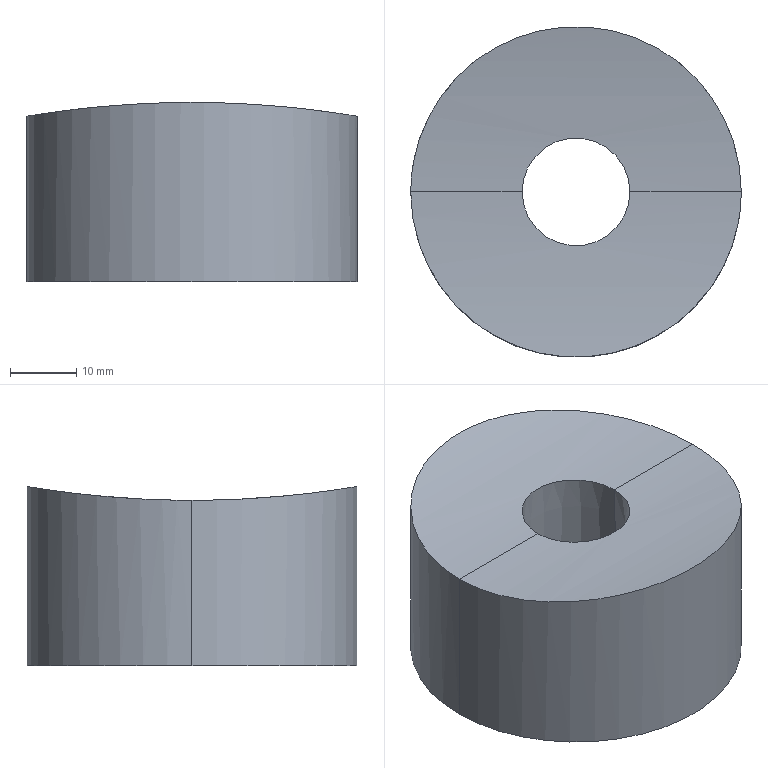Component | SolidWorks | JF21-80.1-1-3(_)-1-SOLID12-1 | 1 solid | 7 faces | box 50 x 50 x 27.1 mm | volume 44357 mm3 | cylinder 4 | cone 2 | plane 1 | commonest cylinder face diameters 300 x2 50 x2
STEP:
#1=CARTESIAN_POINT('',(8.34,-39.37,30.315));
#2=VERTEX_POINT('',#1);
#3=CARTESIAN_POINT('',(8.983,-39.37,30.315));
#4=VERTEX_POINT('',#3);
#5=CARTESIAN_POINT('',(8.34,-39.37,30.315));
#6=CARTESIAN_POINT('',(8.34,-39.391,30.315));
#7=CARTESIAN_POINT('',(8.342,-39.412,30.315));
#8=CARTESIAN_POINT('',(8.348,-39.443,30.315));
#9=CARTESIAN_POINT('',(8.351,-39.453,30.316));
#10=CARTESIAN_POINT('',(8.357,-39.473,30.316));
#11=CARTESIAN_POINT('',(8.361,-39.483,30.316));
#12=CARTESIAN_POINT('',(8.373,-39.512,30.317));
#13=CARTESIAN_POINT('',(8.383,-39.531,30.317));
#14=CARTESIAN_POINT('',(8.406,-39.566,30.318));
#15=CARTESIAN_POINT('',(8.42,-39.582,30.319));
#16=CARTESIAN_POINT('',(8.449,-39.612,30.32));
#17=CARTESIAN_POINT('',(8.465,-39.625,30.32));
#18=CARTESIAN_POINT('',(8.492,-39.643,30.321));
#19=CARTESIAN_POINT('',(8.501,-39.648,30.322));
#20=CARTESIAN_POINT('',(8.519,-39.658,30.322));
#21=CARTESIAN_POINT('',(8.538,-39.667,30.322));
#22=CARTESIAN_POINT('',(8.558,-39.674,30.323));
#23=CARTESIAN_POINT('',(8.578,-39.68,30.323));
#24=CARTESIAN_POINT('',(8.588,-39.683,30.323));
#25=CARTESIAN_POINT('',(8.619,-39.689,30.324));
#26=CARTESIAN_POINT('',(8.64,-39.691,30.324));
#27=CARTESIAN_POINT('',(8.682,-39.691,30.324));
#28=CARTESIAN_POINT('',(8.703,-39.689,30.324));
#29=CARTESIAN_POINT('',(8.745,-39.681,30.323));
#30=CARTESIAN_POINT('',(8.765,-39.675,30.323));
#31=CARTESIAN_POINT('',(8.794,-39.663,30.322));
#32=CARTESIAN_POINT('',(8.803,-39.658,30.322));
#33=CARTESIAN_POINT('',(8.822,-39.648,30.322));
#34=CARTESIAN_POINT('',(8.831,-39.643,30.321));
#35=CARTESIAN_POINT('',(8.857,-39.625,30.32));
#36=CARTESIAN_POINT('',(8.873,-39.612,30.32));
#37=CARTESIAN_POINT('',(8.903,-39.582,30.319));
#38=CARTESIAN_POINT('',(8.917,-39.566,30.318));
#39=CARTESIAN_POINT('',(8.934,-39.54,30.317));
#40=CARTESIAN_POINT('',(8.94,-39.531,30.317));
#41=CARTESIAN_POINT('',(8.95,-39.512,30.317));
#42=CARTESIAN_POINT('',(8.954,-39.503,30.316));
#43=CARTESIAN_POINT('',(8.966,-39.474,30.316));
#44=CARTESIAN_POINT('',(8.972,-39.454,30.316));
#45=CARTESIAN_POINT('',(8.981,-39.413,30.315));
#46=CARTESIAN_POINT('',(8.983,-39.391,30.315));
#47=CARTESIAN_POINT('',(8.983,-39.37,30.315));
#48=B_SPLINE_CURVE_WITH_KNOTS('',3,(#5,#6,#7,#8,#9,#10,#11,#12,#13,#14,#15,#16,#17,#18,#19,#20,#21,#22,#23,#24,#25,#26,#27,#28,#29,#30,#31,#32,#33,#34,#35,#36,#37,#38,#39,#40,#41,#42,#43,#44,#45,#46,#47),.UNSPECIFIED.,.F.,.F.,(4,2,2,2,2,2,2,2,1,2,2,2,2,2,2,2,2,2,2,2,2,4),(0.,0.001594,0.002391,0.003187,0.004781,0.006375,0.007968,0.008765,0.009562,0.01036,0.01116,0.01275,0.01434,0.01594,0.01673,0.01753,0.01912,0.02072,0.02151,0.02231,0.02391,0.0255),.UNSPECIFIED.);
#49=EDGE_CURVE('',#2,#4,#48,.T.);
#50=ORIENTED_EDGE('',*,*,#49,.T.);
#51=CARTESIAN_POINT('',(9.013,-39.37,29.331));
#52=VERTEX_POINT('',#51);
#53=CARTESIAN_POINT('',(9.013,-39.37,29.331));
#54=DIRECTION('',(-0.0312,-0.,0.9995));
#55=VECTOR('',#54,39.37);
#56=LINE('',#53,#55);
#57=EDGE_CURVE('',#52,#4,#56,.T.);
#58=ORIENTED_EDGE('',*,*,#57,.F.);
#59=CARTESIAN_POINT('',(8.309,-39.37,29.331));
#60=VERTEX_POINT('',#59);
#61=CARTESIAN_POINT('',(8.661,-39.37,29.331));
#62=DIRECTION('',(0.,0.,-1.));
#63=DIRECTION('',(-1.,0.,0.));
#64=AXIS2_PLACEMENT_3D('',#61,#62,#63);
#65=CIRCLE('',#64,0.352);
#66=EDGE_CURVE('',#52,#60,#65,.T.);
#67=ORIENTED_EDGE('',*,*,#66,.T.);
#68=CARTESIAN_POINT('',(8.309,-39.37,29.331));
#69=DIRECTION('',(0.0312,0.,0.9995));
#70=VECTOR('',#69,39.37);
#71=LINE('',#68,#70);
#72=EDGE_CURVE('',#60,#2,#71,.T.);
#73=ORIENTED_EDGE('',*,*,#72,.T.);
#74=EDGE_LOOP('',(#50,#58,#67,#73));
#75=FACE_OUTER_BOUND('',#74,.T.);
#76=CARTESIAN_POINT('',(8.661,-39.37,29.331));
#77=DIRECTION('',(0.,0.,-1.));
#78=DIRECTION('',(1.,0.,0.));
#79=AXIS2_PLACEMENT_3D('',#76,#77,#78);
#80=CONICAL_SURFACE('',#79,0.352,0.03121);
#81=ADVANCED_FACE('',(#75),#80,.F.);
#82=CARTESIAN_POINT('',(9.646,-39.37,30.315));
#83=VERTEX_POINT('',#82);
#84=CARTESIAN_POINT('',(7.677,-39.37,30.315));
#85=VERTEX_POINT('',#84);
#86=CARTESIAN_POINT('',(9.646,-39.37,30.315));
#87=CARTESIAN_POINT('',(9.646,-39.305,30.315));
#88=CARTESIAN_POINT('',(9.639,-39.241,30.316));
#89=CARTESIAN_POINT('',(9.62,-39.146,30.319));
#90=CARTESIAN_POINT('',(9.613,-39.115,30.32));
#91=CARTESIAN_POINT('',(9.594,-39.053,30.323));
#92=CARTESIAN_POINT('',(9.583,-39.023,30.325));
#93=CARTESIAN_POINT('',(9.546,-38.933,30.331));
#94=CARTESIAN_POINT('',(9.516,-38.877,30.335));
#95=CARTESIAN_POINT('',(9.471,-38.81,30.342));
#96=CARTESIAN_POINT('',(9.462,-38.797,30.343));
#97=CARTESIAN_POINT('',(9.442,-38.771,30.345));
#98=CARTESIAN_POINT('',(9.432,-38.758,30.347));
#99=CARTESIAN_POINT('',(9.402,-38.721,30.351));
#100=CARTESIAN_POINT('',(9.38,-38.697,30.353));
#101=CARTESIAN_POINT('',(9.312,-38.629,30.361));
#102=CARTESIAN_POINT('',(9.263,-38.588,30.367));
#103=CARTESIAN_POINT('',(9.195,-38.543,30.373));
#104=CARTESIAN_POINT('',(9.182,-38.534,30.374));
#105=CARTESIAN_POINT('',(9.154,-38.518,30.377));
#106=CARTESIAN_POINT('',(9.14,-38.51,30.378));
#107=CARTESIAN_POINT('',(9.097,-38.487,30.381));
#108=CARTESIAN_POINT('',(9.068,-38.473,30.383));
#109=CARTESIAN_POINT('',(9.009,-38.449,30.387));
#110=CARTESIAN_POINT('',(8.979,-38.438,30.389));
#111=CARTESIAN_POINT('',(8.933,-38.424,30.391));
#112=CARTESIAN_POINT('',(8.917,-38.42,30.392));
#113=CARTESIAN_POINT('',(8.886,-38.412,30.393));
#114=CARTESIAN_POINT('',(8.87,-38.408,30.394));
#115=CARTESIAN_POINT('',(8.79,-38.392,30.396));
#116=CARTESIAN_POINT('',(8.726,-38.386,30.398));
#117=CARTESIAN_POINT('',(8.63,-38.386,30.398));
#118=CARTESIAN_POINT('',(8.598,-38.387,30.397));
#119=CARTESIAN_POINT('',(8.549,-38.392,30.397));
#120=CARTESIAN_POINT('',(8.533,-38.394,30.396));
#121=CARTESIAN_POINT('',(8.501,-38.399,30.395));
#122=CARTESIAN_POINT('',(8.485,-38.402,30.395));
#123=CARTESIAN_POINT('',(8.406,-38.417,30.392));
#124=CARTESIAN_POINT('',(8.345,-38.436,30.389));
#125=CARTESIAN_POINT('',(8.255,-38.473,30.383));
#126=CARTESIAN_POINT('',(8.226,-38.487,30.381));
#127=CARTESIAN_POINT('',(8.169,-38.517,30.377));
#128=CARTESIAN_POINT('',(8.141,-38.534,30.374));
#129=CARTESIAN_POINT('',(8.088,-38.569,30.369));
#130=CARTESIAN_POINT('',(8.062,-38.588,30.367));
#131=CARTESIAN_POINT('',(8.013,-38.629,30.362));
#132=CARTESIAN_POINT('',(7.989,-38.651,30.359));
#133=CARTESIAN_POINT('',(7.92,-38.719,30.351));
#134=CARTESIAN_POINT('',(7.879,-38.769,30.345));
#135=CARTESIAN_POINT('',(7.826,-38.849,30.338));
#136=CARTESIAN_POINT('',(7.809,-38.876,30.336));
#137=CARTESIAN_POINT('',(7.786,-38.919,30.332));
#138=CARTESIAN_POINT('',(7.779,-38.934,30.331));
#139=CARTESIAN_POINT('',(7.765,-38.963,30.329));
#140=CARTESIAN_POINT('',(7.759,-38.978,30.328));
#141=CARTESIAN_POINT('',(7.728,-39.052,30.323));
#142=CARTESIAN_POINT('',(7.709,-39.113,30.32));
#143=CARTESIAN_POINT('',(7.69,-39.208,30.317));
#144=CARTESIAN_POINT('',(7.685,-39.24,30.316));
#145=CARTESIAN_POINT('',(7.679,-39.305,30.315));
#146=CARTESIAN_POINT('',(7.677,-39.338,30.315));
#147=CARTESIAN_POINT('',(7.677,-39.37,30.315));
#148=B_SPLINE_CURVE_WITH_KNOTS('',3,(#86,#87,#88,#89,#90,#91,#92,#93,#94,#95,#96,#97,#98,#99,#100,#101,#102,#103,#104,#105,#106,#107,#108,#109,#110,#111,#112,#113,#114,#115,#116,#117,#118,#119,#120,#121,#122,#123,#124,#125,#126,#127,#128,#129,#130,#131,#132,#133,#134,#135,#136,#137,#138,#139,#140,#141,#142,#143,#144,#145,#146,#147),.UNSPECIFIED.,.F.,.F.,(4,2,2,2,2,2,2,2,2,2,2,2,2,2,2,2,2,2,2,2,2,2,2,2,2,2,2,2,2,2,4),(0.,0.004892,0.007339,0.009785,0.01468,0.0159,0.01712,0.01957,0.02446,0.02569,0.02691,0.02935,0.0318,0.03302,0.03425,0.03914,0.04159,0.04281,0.04403,0.04892,0.05137,0.05382,0.05626,0.05871,0.0636,0.06605,0.06727,0.06849,0.07339,0.07583,0.07828),.UNSPECIFIED.);
#149=EDGE_CURVE('',#83,#85,#148,.T.);
#150=ORIENTED_EDGE('',*,*,#149,.T.);
#151=CARTESIAN_POINT('',(-15.748,-39.37,30.315));
#152=DIRECTION('',(1.,0.,0.));
#153=VECTOR('',#152,39.37);
#154=LINE('',#151,#153);
#155=EDGE_CURVE('',#85,#2,#154,.T.);
#156=ORIENTED_EDGE('',*,*,#155,.T.);
#157=CARTESIAN_POINT('',(8.983,-39.37,30.315));
#158=CARTESIAN_POINT('',(8.983,-39.349,30.315));
#159=CARTESIAN_POINT('',(8.981,-39.328,30.315));
#160=CARTESIAN_POINT('',(8.974,-39.297,30.315));
#161=CARTESIAN_POINT('',(8.972,-39.287,30.316));
#162=CARTESIAN_POINT('',(8.966,-39.267,30.316));
#163=CARTESIAN_POINT('',(8.962,-39.257,30.316));
#164=CARTESIAN_POINT('',(8.95,-39.228,30.317));
#165=CARTESIAN_POINT('',(8.94,-39.209,30.317));
#166=CARTESIAN_POINT('',(8.917,-39.174,30.318));
#167=CARTESIAN_POINT('',(8.903,-39.158,30.319));
#168=CARTESIAN_POINT('',(8.874,-39.128,30.32));
#169=CARTESIAN_POINT('',(8.858,-39.115,30.32));
#170=CARTESIAN_POINT('',(8.831,-39.097,30.321));
#171=CARTESIAN_POINT('',(8.822,-39.092,30.322));
#172=CARTESIAN_POINT('',(8.804,-39.082,30.322));
#173=CARTESIAN_POINT('',(8.785,-39.073,30.322));
#174=CARTESIAN_POINT('',(8.765,-39.066,30.323));
#175=CARTESIAN_POINT('',(8.745,-39.06,30.323));
#176=CARTESIAN_POINT('',(8.734,-39.057,30.323));
#177=CARTESIAN_POINT('',(8.703,-39.051,30.324));
#178=CARTESIAN_POINT('',(8.683,-39.049,30.324));
#179=CARTESIAN_POINT('',(8.641,-39.049,30.324));
#180=CARTESIAN_POINT('',(8.619,-39.051,30.324));
#181=CARTESIAN_POINT('',(8.578,-39.059,30.323));
#182=CARTESIAN_POINT('',(8.558,-39.065,30.323));
#183=CARTESIAN_POINT('',(8.529,-39.077,30.322));
#184=CARTESIAN_POINT('',(8.519,-39.082,30.322));
#185=CARTESIAN_POINT('',(8.501,-39.092,30.322));
#186=CARTESIAN_POINT('',(8.492,-39.097,30.321));
#187=CARTESIAN_POINT('',(8.466,-39.115,30.32));
#188=CARTESIAN_POINT('',(8.449,-39.128,30.32));
#189=CARTESIAN_POINT('',(8.419,-39.158,30.319));
#190=CARTESIAN_POINT('',(8.406,-39.174,30.318));
#191=CARTESIAN_POINT('',(8.389,-39.2,30.317));
#192=CARTESIAN_POINT('',(8.383,-39.209,30.317));
#193=CARTESIAN_POINT('',(8.373,-39.228,30.317));
#194=CARTESIAN_POINT('',(8.369,-39.237,30.316));
#195=CARTESIAN_POINT('',(8.357,-39.266,30.316));
#196=CARTESIAN_POINT('',(8.351,-39.286,30.316));
#197=CARTESIAN_POINT('',(8.342,-39.328,30.315));
#198=CARTESIAN_POINT('',(8.34,-39.349,30.315));
#199=CARTESIAN_POINT('',(8.34,-39.37,30.315));
#200=B_SPLINE_CURVE_WITH_KNOTS('',3,(#157,#158,#159,#160,#161,#162,#163,#164,#165,#166,#167,#168,#169,#170,#171,#172,#173,#174,#175,#176,#177,#178,#179,#180,#181,#182,#183,#184,#185,#186,#187,#188,#189,#190,#191,#192,#193,#194,#195,#196,#197,#198,#199),.UNSPECIFIED.,.F.,.F.,(4,2,2,2,2,2,2,2,1,2,2,2,2,2,2,2,2,2,2,2,2,4),(0.,0.001594,0.002391,0.003187,0.004781,0.006375,0.007968,0.008765,0.009562,0.01036,0.01116,0.01275,0.01434,0.01594,0.01673,0.01753,0.01912,0.02072,0.02151,0.02231,0.02391,0.0255),.UNSPECIFIED.);
#201=EDGE_CURVE('',#4,#2,#200,.T.);
#202=ORIENTED_EDGE('',*,*,#201,.F.);
#203=CARTESIAN_POINT('',(-15.748,-39.37,30.315));
#204=DIRECTION('',(1.,0.,0.));
#205=VECTOR('',#204,39.37);
#206=LINE('',#203,#205);
#207=EDGE_CURVE('',#4,#83,#206,.T.);
#208=ORIENTED_EDGE('',*,*,#207,.T.);
#209=EDGE_LOOP('',(#150,#156,#202,#208));
#210=FACE_OUTER_BOUND('',#209,.T.);
#211=CARTESIAN_POINT('',(-15.748,-39.37,36.22));
#212=DIRECTION('',(1.,0.,0.));
#213=DIRECTION('',(0.,0.,1.));
#214=AXIS2_PLACEMENT_3D('',#211,#212,#213);
#215=CYLINDRICAL_SURFACE('',#214,5.906);
#216=ADVANCED_FACE('',(#210),#215,.F.);
#217=ORIENTED_EDGE('',*,*,#149,.F.);
#218=CARTESIAN_POINT('',(9.646,-39.37,29.331));
#219=VERTEX_POINT('',#218);
#220=CARTESIAN_POINT('',(9.646,-39.37,30.709));
#221=DIRECTION('',(0.,0.,1.));
#222=VECTOR('',#221,39.37);
#223=LINE('',#220,#222);
#224=EDGE_CURVE('',#219,#83,#223,.T.);
#225=ORIENTED_EDGE('',*,*,#224,.F.);
#226=CARTESIAN_POINT('',(7.677,-39.37,29.331));
#227=VERTEX_POINT('',#226);
#228=CARTESIAN_POINT('',(8.661,-39.37,29.331));
#229=DIRECTION('',(0.,0.,1.));
#230=DIRECTION('',(1.,0.,0.));
#231=AXIS2_PLACEMENT_3D('',#228,#229,#230);
#232=CIRCLE('',#231,0.9843);
#233=EDGE_CURVE('',#219,#227,#232,.T.);
#234=ORIENTED_EDGE('',*,*,#233,.T.);
#235=CARTESIAN_POINT('',(7.677,-39.37,30.709));
#236=DIRECTION('',(0.,0.,1.));
#237=VECTOR('',#236,39.37);
#238=LINE('',#235,#237);
#239=EDGE_CURVE('',#227,#85,#238,.T.);
#240=ORIENTED_EDGE('',*,*,#239,.T.);
#241=EDGE_LOOP('',(#217,#225,#234,#240));
#242=FACE_OUTER_BOUND('',#241,.T.);
#243=CARTESIAN_POINT('',(8.661,-39.37,30.709));
#244=DIRECTION('',(0.,0.,-1.));
#245=DIRECTION('',(1.,0.,0.));
#246=AXIS2_PLACEMENT_3D('',#243,#244,#245);
#247=CYLINDRICAL_SURFACE('',#246,0.9843);
#248=ADVANCED_FACE('',(#242),#247,.T.);
#249=ORIENTED_EDGE('',*,*,#224,.T.);
#250=CARTESIAN_POINT('',(7.677,-39.37,30.315));
#251=CARTESIAN_POINT('',(7.677,-39.435,30.315));
#252=CARTESIAN_POINT('',(7.684,-39.499,30.316));
#253=CARTESIAN_POINT('',(7.702,-39.594,30.319));
#254=CARTESIAN_POINT('',(7.71,-39.625,30.32));
#255=CARTESIAN_POINT('',(7.729,-39.687,30.323));
#256=CARTESIAN_POINT('',(7.74,-39.718,30.325));
#257=CARTESIAN_POINT('',(7.777,-39.807,30.331));
#258=CARTESIAN_POINT('',(7.807,-39.863,30.335));
#259=CARTESIAN_POINT('',(7.852,-39.93,30.342));
#260=CARTESIAN_POINT('',(7.861,-39.943,30.343));
#261=CARTESIAN_POINT('',(7.88,-39.969,30.345));
#262=CARTESIAN_POINT('',(7.89,-39.982,30.347));
#263=CARTESIAN_POINT('',(7.921,-40.02,30.351));
#264=CARTESIAN_POINT('',(7.943,-40.043,30.353));
#265=CARTESIAN_POINT('',(8.011,-40.111,30.361));
#266=CARTESIAN_POINT('',(8.06,-40.152,30.367));
#267=CARTESIAN_POINT('',(8.127,-40.197,30.373));
#268=CARTESIAN_POINT('',(8.141,-40.206,30.374));
#269=CARTESIAN_POINT('',(8.169,-40.222,30.377));
#270=CARTESIAN_POINT('',(8.183,-40.23,30.378));
#271=CARTESIAN_POINT('',(8.225,-40.253,30.381));
#272=CARTESIAN_POINT('',(8.254,-40.267,30.383));
#273=CARTESIAN_POINT('',(8.314,-40.291,30.387));
#274=CARTESIAN_POINT('',(8.344,-40.302,30.389));
#275=CARTESIAN_POINT('',(8.39,-40.316,30.391));
#276=CARTESIAN_POINT('',(8.406,-40.321,30.392));
#277=CARTESIAN_POINT('',(8.437,-40.329,30.393));
#278=CARTESIAN_POINT('',(8.453,-40.332,30.394));
#279=CARTESIAN_POINT('',(8.532,-40.348,30.396));
#280=CARTESIAN_POINT('',(8.596,-40.354,30.398));
#281=CARTESIAN_POINT('',(8.693,-40.354,30.398));
#282=CARTESIAN_POINT('',(8.725,-40.353,30.397));
#283=CARTESIAN_POINT('',(8.774,-40.348,30.397));
#284=CARTESIAN_POINT('',(8.79,-40.346,30.396));
#285=CARTESIAN_POINT('',(8.822,-40.341,30.395));
#286=CARTESIAN_POINT('',(8.838,-40.339,30.395));
#287=CARTESIAN_POINT('',(8.917,-40.323,30.392));
#288=CARTESIAN_POINT('',(8.978,-40.304,30.389));
#289=CARTESIAN_POINT('',(9.067,-40.267,30.383));
#290=CARTESIAN_POINT('',(9.097,-40.253,30.381));
#291=CARTESIAN_POINT('',(9.154,-40.223,30.377));
#292=CARTESIAN_POINT('',(9.181,-40.206,30.374));
#293=CARTESIAN_POINT('',(9.235,-40.171,30.369));
#294=CARTESIAN_POINT('',(9.26,-40.152,30.367));
#295=CARTESIAN_POINT('',(9.31,-40.111,30.362));
#296=CARTESIAN_POINT('',(9.334,-40.089,30.359));
#297=CARTESIAN_POINT('',(9.403,-40.021,30.351));
#298=CARTESIAN_POINT('',(9.443,-39.971,30.345));
#299=CARTESIAN_POINT('',(9.497,-39.891,30.338));
#300=CARTESIAN_POINT('',(9.514,-39.864,30.336));
#301=CARTESIAN_POINT('',(9.536,-39.821,30.332));
#302=CARTESIAN_POINT('',(9.544,-39.807,30.331));
#303=CARTESIAN_POINT('',(9.558,-39.777,30.329));
#304=CARTESIAN_POINT('',(9.564,-39.762,30.328));
#305=CARTESIAN_POINT('',(9.595,-39.688,30.323));
#306=CARTESIAN_POINT('',(9.614,-39.627,30.32));
#307=CARTESIAN_POINT('',(9.633,-39.532,30.317));
#308=CARTESIAN_POINT('',(9.638,-39.5,30.316));
#309=CARTESIAN_POINT('',(9.644,-39.435,30.315));
#310=CARTESIAN_POINT('',(9.646,-39.403,30.315));
#311=CARTESIAN_POINT('',(9.646,-39.37,30.315));
#312=B_SPLINE_CURVE_WITH_KNOTS('',3,(#250,#251,#252,#253,#254,#255,#256,#257,#258,#259,#260,#261,#262,#263,#264,#265,#266,#267,#268,#269,#270,#271,#272,#273,#274,#275,#276,#277,#278,#279,#280,#281,#282,#283,#284,#285,#286,#287,#288,#289,#290,#291,#292,#293,#294,#295,#296,#297,#298,#299,#300,#301,#302,#303,#304,#305,#306,#307,#308,#309,#310,#311),.UNSPECIFIED.,.F.,.F.,(4,2,2,2,2,2,2,2,2,2,2,2,2,2,2,2,2,2,2,2,2,2,2,2,2,2,2,2,2,2,4),(0.,0.004892,0.007339,0.009785,0.01468,0.0159,0.01712,0.01957,0.02446,0.02569,0.02691,0.02935,0.0318,0.03302,0.03425,0.03914,0.04159,0.04281,0.04403,0.04892,0.05137,0.05382,0.05626,0.05871,0.0636,0.06605,0.06727,0.06849,0.07339,0.07583,0.07828),.UNSPECIFIED.);
#313=EDGE_CURVE('',#85,#83,#312,.T.);
#314=ORIENTED_EDGE('',*,*,#313,.F.);
#315=ORIENTED_EDGE('',*,*,#239,.F.);
#316=CARTESIAN_POINT('',(8.661,-39.37,29.331));
#317=DIRECTION('',(0.,0.,1.));
#318=DIRECTION('',(1.,0.,0.));
#319=AXIS2_PLACEMENT_3D('',#316,#317,#318);
#320=CIRCLE('',#319,0.9843);
#321=EDGE_CURVE('',#227,#219,#320,.T.);
#322=ORIENTED_EDGE('',*,*,#321,.T.);
#323=EDGE_LOOP('',(#249,#314,#315,#322));
#324=FACE_OUTER_BOUND('',#323,.T.);
#325=CARTESIAN_POINT('',(8.661,-39.37,30.709));
#326=DIRECTION('',(0.,0.,-1.));
#327=DIRECTION('',(1.,0.,0.));
#328=AXIS2_PLACEMENT_3D('',#325,#326,#327);
#329=CYLINDRICAL_SURFACE('',#328,0.9843);
#330=ADVANCED_FACE('',(#324),#329,.T.);
#331=CARTESIAN_POINT('',(8.661,-39.37,29.331));
#332=DIRECTION('',(0.,0.,-1.));
#333=DIRECTION('',(-1.,0.,0.));
#334=AXIS2_PLACEMENT_3D('',#331,#332,#333);
#335=CIRCLE('',#334,0.352);
#336=EDGE_CURVE('',#60,#52,#335,.T.);
#337=ORIENTED_EDGE('',*,*,#336,.F.);
#338=ORIENTED_EDGE('',*,*,#66,.F.);
#339=EDGE_LOOP('',(#337,#338));
#340=FACE_BOUND('',#339,.T.);
#341=ORIENTED_EDGE('',*,*,#321,.F.);
#342=ORIENTED_EDGE('',*,*,#233,.F.);
#343=EDGE_LOOP('',(#341,#342));
#344=FACE_OUTER_BOUND('',#343,.T.);
#345=CARTESIAN_POINT('',(8.661,-39.37,29.331));
#346=DIRECTION('',(0.,0.,1.));
#347=DIRECTION('',(-1.,0.,0.));
#348=AXIS2_PLACEMENT_3D('',#345,#346,#347);
#349=PLANE('',#348);
#350=ADVANCED_FACE('',(#340,#344),#349,.F.);
#351=ORIENTED_EDGE('',*,*,#155,.F.);
#352=ORIENTED_EDGE('',*,*,#313,.T.);
#353=ORIENTED_EDGE('',*,*,#207,.F.);
#354=ORIENTED_EDGE('',*,*,#49,.F.);
#355=EDGE_LOOP('',(#351,#352,#353,#354));
#356=FACE_OUTER_BOUND('',#355,.T.);
#357=CARTESIAN_POINT('',(-15.748,-39.37,36.22));
#358=DIRECTION('',(1.,0.,0.));
#359=DIRECTION('',(0.,0.,1.));
#360=AXIS2_PLACEMENT_3D('',#357,#358,#359);
#361=CYLINDRICAL_SURFACE('',#360,5.906);
#362=ADVANCED_FACE('',(#356),#361,.F.);
#363=ORIENTED_EDGE('',*,*,#57,.T.);
#364=ORIENTED_EDGE('',*,*,#201,.T.);
#365=ORIENTED_EDGE('',*,*,#72,.F.);
#366=ORIENTED_EDGE('',*,*,#336,.T.);
#367=EDGE_LOOP('',(#363,#364,#365,#366));
#368=FACE_OUTER_BOUND('',#367,.T.);
#369=CARTESIAN_POINT('',(8.661,-39.37,29.331));
#370=DIRECTION('',(0.,0.,-1.));
#371=DIRECTION('',(1.,0.,0.));
#372=AXIS2_PLACEMENT_3D('',#369,#370,#371);
#373=CONICAL_SURFACE('',#372,0.352,0.03121);
#374=ADVANCED_FACE('',(#368),#373,.F.);
#375=CLOSED_SHELL('',(#81,#216,#248,#330,#350,#362,#374));
#376=MANIFOLD_SOLID_BREP('',#375);
#377=CARTESIAN_POINT('',(0.,0.,0.));
#378=DIRECTION('',(0.,0.,1.));
#379=DIRECTION('',(1.,0.,0.));
#380=AXIS2_PLACEMENT_3D('',#377,#378,#379);
#381=(LENGTH_UNIT()NAMED_UNIT(*)SI_UNIT($,.METRE.));
#382=LENGTH_MEASURE_WITH_UNIT(LENGTH_MEASURE(0.0254),#381);
#383=DIMENSIONAL_EXPONENTS(1.,0.,0.,0.,0.,0.,0.);
#384=(CONVERSION_BASED_UNIT('',#382)LENGTH_UNIT()NAMED_UNIT(#383));
#385=UNCERTAINTY_MEASURE_WITH_UNIT(LENGTH_MEASURE(0.00001),#384,'','');
#386=(NAMED_UNIT(*)PLANE_ANGLE_UNIT()SI_UNIT($,.RADIAN.));
#387=(NAMED_UNIT(*)SI_UNIT($,.STERADIAN.)SOLID_ANGLE_UNIT());
#388=(GEOMETRIC_REPRESENTATION_CONTEXT(3)GLOBAL_UNCERTAINTY_ASSIGNED_CONTEXT((#385))GLOBAL_UNIT_ASSIGNED_CONTEXT((#384,#386,#387))REPRESENTATION_CONTEXT('',''));
#389=ADVANCED_BREP_SHAPE_REPRESENTATION('',(#376,#380),#388);
#390=COLOUR_RGB('',0.7922,0.8196,0.9333);
#391=FILL_AREA_STYLE_COLOUR('',#390);
#392=FILL_AREA_STYLE('',(#391));
#393=SURFACE_STYLE_FILL_AREA(#392);
#394=SURFACE_SIDE_STYLE('',(#393));
#395=SURFACE_STYLE_USAGE(.BOTH.,#394);
#396=PRESENTATION_STYLE_ASSIGNMENT((#395));
#397=STYLED_ITEM('',(#396),#376);
#398=PRESENTATION_LAYER_ASSIGNMENT('','',(#397));
#399=(LENGTH_UNIT()NAMED_UNIT(*)SI_UNIT($,.METRE.));
#400=LENGTH_MEASURE_WITH_UNIT(LENGTH_MEASURE(0.0254),#399);
#401=DIMENSIONAL_EXPONENTS(1.,0.,0.,0.,0.,0.,0.);
#402=(CONVERSION_BASED_UNIT('',#400)LENGTH_UNIT()NAMED_UNIT(#401));
#403=UNCERTAINTY_MEASURE_WITH_UNIT(LENGTH_MEASURE(0.00001),#402,'','');
#404=(NAMED_UNIT(*)PLANE_ANGLE_UNIT()SI_UNIT($,.RADIAN.));
#405=(NAMED_UNIT(*)SI_UNIT($,.STERADIAN.)SOLID_ANGLE_UNIT());
#406=(GEOMETRIC_REPRESENTATION_CONTEXT(3)GLOBAL_UNCERTAINTY_ASSIGNED_CONTEXT((#403))GLOBAL_UNIT_ASSIGNED_CONTEXT((#402,#404,#405))REPRESENTATION_CONTEXT('',''));
#407=MECHANICAL_DESIGN_GEOMETRIC_PRESENTATION_REPRESENTATION('',(#397),#406);